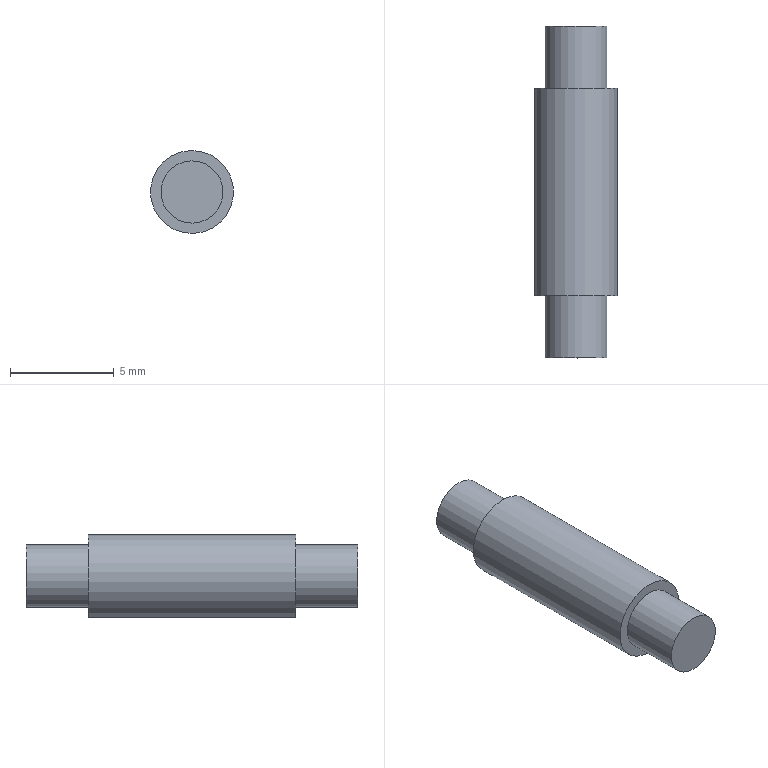Component | NX | CONNECTING_PIN_2_2 | 1 solid | 7 faces | box 4 x 16 x 4 mm | volume 168 mm3 | plane 4 | cylinder 3 | commonest cylinder face diameters 3 x2 4 x1
STEP:
#1=CARTESIAN_POINT('',(0.,0.,0.));
#2=DIRECTION('',(0.,0.,1.));
#3=DIRECTION('',(1.,0.,0.));
#4=AXIS2_PLACEMENT_3D('',#1,#2,#3);
#5=CARTESIAN_POINT('',(-75.879,-51.,18.369));
#6=VERTEX_POINT('',#5);
#7=CARTESIAN_POINT('',(-77.374,-51.,18.5));
#8=DIRECTION('',(0.,-1.,-0.));
#9=DIRECTION('',(0.9962,0.,-0.08716));
#10=AXIS2_PLACEMENT_3D('',#7,#8,#9);
#11=CIRCLE('',#10,1.5);
#12=CARTESIAN_POINT('',(-77.374,-51.,18.5));
#13=DIRECTION('',(0.,1.,0.));
#14=DIRECTION('',(-0.9962,-0.,0.08716));
#15=AXIS2_PLACEMENT_3D('',#12,#13,#14);
#16=PLANE('',#15);
#17=CARTESIAN_POINT('',(-1.5,-0.));
#18=CARTESIAN_POINT('',(-1.5,2.598));
#19=CARTESIAN_POINT('',(0.75,1.299));
#20=CARTESIAN_POINT('',(3.,0.));
#21=CARTESIAN_POINT('',(0.75,-1.299));
#22=CARTESIAN_POINT('',(-1.5,-2.598));
#23=CARTESIAN_POINT('',(-1.5,-0.));
#24=(BOUNDED_CURVE()B_SPLINE_CURVE(2,(#17,#18,#19,#20,#21,#22,#23),.UNSPECIFIED.,.T.,.F.)B_SPLINE_CURVE_WITH_KNOTS((1,2,2,2,2,1),(-2.094,0.,2.094,4.189,6.283,8.378),.UNSPECIFIED.)CURVE()GEOMETRIC_REPRESENTATION_ITEM()RATIONAL_B_SPLINE_CURVE((1.,0.5,1.,0.5,1.,0.5,1.))REPRESENTATION_ITEM(''));
#25=(GEOMETRIC_REPRESENTATION_CONTEXT(2)PARAMETRIC_REPRESENTATION_CONTEXT()REPRESENTATION_CONTEXT('',''));
#26=DEFINITIONAL_REPRESENTATION('',(#24),#25);
#27=PCURVE('',#16,#26);
#28=CARTESIAN_POINT('',(-77.374,-51.,18.5));
#29=DIRECTION('',(0.,-1.,-0.));
#30=DIRECTION('',(0.9962,0.,-0.08716));
#31=AXIS2_PLACEMENT_3D('',#28,#29,#30);
#32=CYLINDRICAL_SURFACE('',#31,1.5);
#33=CARTESIAN_POINT('',(0.,0.));
#34=DIRECTION('',(1.,0.));
#35=VECTOR('',#34,1.);
#36=LINE('',#33,#35);
#37=(GEOMETRIC_REPRESENTATION_CONTEXT(2)PARAMETRIC_REPRESENTATION_CONTEXT()REPRESENTATION_CONTEXT('',''));
#38=DEFINITIONAL_REPRESENTATION('',(#36),#37);
#39=PCURVE('',#32,#38);
#40=SURFACE_CURVE('',#11,(#27,#39),.PCURVE_S1.);
#41=EDGE_CURVE('',#6,#6,#40,.T.);
#42=ORIENTED_EDGE('',*,*,#41,.F.);
#43=EDGE_LOOP('',(#42));
#44=FACE_BOUND('',#43,.T.);
#45=ADVANCED_FACE('',(#44),#16,.T.);
#46=CARTESIAN_POINT('',(-75.879,-54.,18.369));
#47=VERTEX_POINT('',#46);
#48=CARTESIAN_POINT('',(-77.374,-54.,18.5));
#49=DIRECTION('',(-0.,1.,0.));
#50=DIRECTION('',(0.9962,0.,-0.08716));
#51=AXIS2_PLACEMENT_3D('',#48,#49,#50);
#52=CIRCLE('',#51,1.5);
#53=CARTESIAN_POINT('',(6.283,3.));
#54=DIRECTION('',(-1.,0.));
#55=VECTOR('',#54,1.);
#56=LINE('',#53,#55);
#57=(GEOMETRIC_REPRESENTATION_CONTEXT(2)PARAMETRIC_REPRESENTATION_CONTEXT()REPRESENTATION_CONTEXT('',''));
#58=DEFINITIONAL_REPRESENTATION('',(#56),#57);
#59=PCURVE('',#32,#58);
#60=CARTESIAN_POINT('',(-77.374,-54.,18.5));
#61=DIRECTION('',(0.,1.,0.));
#62=DIRECTION('',(-0.9962,-0.,0.08716));
#63=AXIS2_PLACEMENT_3D('',#60,#61,#62);
#64=PLANE('',#63);
#65=CARTESIAN_POINT('',(0.,0.));
#66=DIRECTION('',(-1.,-0.));
#67=AXIS2_PLACEMENT_2D('',#65,#66);
#68=CIRCLE('',#67,1.5);
#69=(GEOMETRIC_REPRESENTATION_CONTEXT(2)PARAMETRIC_REPRESENTATION_CONTEXT()REPRESENTATION_CONTEXT('',''));
#70=DEFINITIONAL_REPRESENTATION('',(#68),#69);
#71=PCURVE('',#64,#70);
#72=SURFACE_CURVE('',#52,(#59,#71),.PCURVE_S1.);
#73=EDGE_CURVE('',#47,#47,#72,.T.);
#74=ORIENTED_EDGE('',*,*,#73,.T.);
#75=CARTESIAN_POINT('',(-75.879,-51.,18.369));
#76=CARTESIAN_POINT('',(-75.879,-54.,18.369));
#77=B_SPLINE_CURVE_WITH_KNOTS('',1,(#75,#76),.UNSPECIFIED.,.F.,.F.,(2,2),(0.,3.),.PIECEWISE_BEZIER_KNOTS.);
#78=CARTESIAN_POINT('',(0.,0.));
#79=DIRECTION('',(0.,1.));
#80=VECTOR('',#79,1.);
#81=LINE('',#78,#80);
#82=(GEOMETRIC_REPRESENTATION_CONTEXT(2)PARAMETRIC_REPRESENTATION_CONTEXT()REPRESENTATION_CONTEXT('',''));
#83=DEFINITIONAL_REPRESENTATION('',(#81),#82);
#84=PCURVE('',#32,#83);
#85=CARTESIAN_POINT('',(6.283,0.));
#86=DIRECTION('',(0.,1.));
#87=VECTOR('',#86,1.);
#88=LINE('',#85,#87);
#89=(GEOMETRIC_REPRESENTATION_CONTEXT(2)PARAMETRIC_REPRESENTATION_CONTEXT()REPRESENTATION_CONTEXT('',''));
#90=DEFINITIONAL_REPRESENTATION('',(#88),#89);
#91=PCURVE('',#32,#90);
#92=SEAM_CURVE('',#77,(#84,#91),.PCURVE_S1.);
#93=EDGE_CURVE('',#6,#47,#92,.T.);
#94=ORIENTED_EDGE('',*,*,#93,.F.);
#95=ORIENTED_EDGE('',*,*,#41,.T.);
#96=ORIENTED_EDGE('',*,*,#93,.T.);
#97=EDGE_LOOP('',(#74,#94,#95,#96));
#98=FACE_BOUND('',#97,.T.);
#99=ADVANCED_FACE('',(#98),#32,.T.);
#100=CARTESIAN_POINT('',(-75.879,-64.,18.369));
#101=VERTEX_POINT('',#100);
#102=CARTESIAN_POINT('',(-77.374,-64.,18.5));
#103=DIRECTION('',(0.,-1.,-0.));
#104=DIRECTION('',(0.9962,0.,-0.08716));
#105=AXIS2_PLACEMENT_3D('',#102,#103,#104);
#106=CIRCLE('',#105,1.5);
#107=CARTESIAN_POINT('',(-77.374,-64.,18.5));
#108=DIRECTION('',(0.,-1.,-0.));
#109=DIRECTION('',(0.9962,0.,-0.08716));
#110=AXIS2_PLACEMENT_3D('',#107,#108,#109);
#111=PLANE('',#110);
#112=CARTESIAN_POINT('',(0.,0.));
#113=DIRECTION('',(1.,-0.));
#114=AXIS2_PLACEMENT_2D('',#112,#113);
#115=CIRCLE('',#114,1.5);
#116=(GEOMETRIC_REPRESENTATION_CONTEXT(2)PARAMETRIC_REPRESENTATION_CONTEXT()REPRESENTATION_CONTEXT('',''));
#117=DEFINITIONAL_REPRESENTATION('',(#115),#116);
#118=PCURVE('',#111,#117);
#119=CARTESIAN_POINT('',(-77.374,-64.,18.5));
#120=DIRECTION('',(0.,-1.,-0.));
#121=DIRECTION('',(0.9962,0.,-0.08716));
#122=AXIS2_PLACEMENT_3D('',#119,#120,#121);
#123=CYLINDRICAL_SURFACE('',#122,1.5);
#124=CARTESIAN_POINT('',(0.,0.));
#125=DIRECTION('',(1.,0.));
#126=VECTOR('',#125,1.);
#127=LINE('',#124,#126);
#128=(GEOMETRIC_REPRESENTATION_CONTEXT(2)PARAMETRIC_REPRESENTATION_CONTEXT()REPRESENTATION_CONTEXT('',''));
#129=DEFINITIONAL_REPRESENTATION('',(#127),#128);
#130=PCURVE('',#123,#129);
#131=SURFACE_CURVE('',#106,(#118,#130),.PCURVE_S1.);
#132=EDGE_CURVE('',#101,#101,#131,.T.);
#133=ORIENTED_EDGE('',*,*,#132,.F.);
#134=EDGE_LOOP('',(#133));
#135=FACE_BOUND('',#134,.T.);
#136=CARTESIAN_POINT('',(-75.381,-64.,18.326));
#137=VERTEX_POINT('',#136);
#138=CARTESIAN_POINT('',(-77.374,-64.,18.5));
#139=DIRECTION('',(0.,-1.,-0.));
#140=DIRECTION('',(0.9962,0.,-0.08716));
#141=AXIS2_PLACEMENT_3D('',#138,#139,#140);
#142=CIRCLE('',#141,2.);
#143=CARTESIAN_POINT('',(0.,0.));
#144=DIRECTION('',(1.,-0.));
#145=AXIS2_PLACEMENT_2D('',#143,#144);
#146=CIRCLE('',#145,2.);
#147=(GEOMETRIC_REPRESENTATION_CONTEXT(2)PARAMETRIC_REPRESENTATION_CONTEXT()REPRESENTATION_CONTEXT('',''));
#148=DEFINITIONAL_REPRESENTATION('',(#146),#147);
#149=PCURVE('',#111,#148);
#150=CARTESIAN_POINT('',(-77.374,-54.,18.5));
#151=DIRECTION('',(0.,-1.,-0.));
#152=DIRECTION('',(0.9962,0.,-0.08716));
#153=AXIS2_PLACEMENT_3D('',#150,#151,#152);
#154=CYLINDRICAL_SURFACE('',#153,2.);
#155=CARTESIAN_POINT('',(0.,10.));
#156=DIRECTION('',(1.,0.));
#157=VECTOR('',#156,1.);
#158=LINE('',#155,#157);
#159=(GEOMETRIC_REPRESENTATION_CONTEXT(2)PARAMETRIC_REPRESENTATION_CONTEXT()REPRESENTATION_CONTEXT('',''));
#160=DEFINITIONAL_REPRESENTATION('',(#158),#159);
#161=PCURVE('',#154,#160);
#162=SURFACE_CURVE('',#142,(#149,#161),.PCURVE_S1.);
#163=EDGE_CURVE('',#137,#137,#162,.T.);
#164=ORIENTED_EDGE('',*,*,#163,.T.);
#165=EDGE_LOOP('',(#164));
#166=FACE_BOUND('',#165,.T.);
#167=ADVANCED_FACE('',(#135,#166),#111,.T.);
#168=ORIENTED_EDGE('',*,*,#73,.F.);
#169=EDGE_LOOP('',(#168));
#170=FACE_BOUND('',#169,.T.);
#171=CARTESIAN_POINT('',(-75.381,-54.,18.326));
#172=VERTEX_POINT('',#171);
#173=CARTESIAN_POINT('',(-77.374,-54.,18.5));
#174=DIRECTION('',(0.,-1.,-0.));
#175=DIRECTION('',(0.9962,0.,-0.08716));
#176=AXIS2_PLACEMENT_3D('',#173,#174,#175);
#177=CIRCLE('',#176,2.);
#178=CARTESIAN_POINT('',(-2.,-0.));
#179=CARTESIAN_POINT('',(-2.,3.464));
#180=CARTESIAN_POINT('',(1.,1.732));
#181=CARTESIAN_POINT('',(4.,0.));
#182=CARTESIAN_POINT('',(1.,-1.732));
#183=CARTESIAN_POINT('',(-2.,-3.464));
#184=CARTESIAN_POINT('',(-2.,-0.));
#185=(BOUNDED_CURVE()B_SPLINE_CURVE(2,(#178,#179,#180,#181,#182,#183,#184),.UNSPECIFIED.,.T.,.F.)B_SPLINE_CURVE_WITH_KNOTS((1,2,2,2,2,1),(-2.094,0.,2.094,4.189,6.283,8.378),.UNSPECIFIED.)CURVE()GEOMETRIC_REPRESENTATION_ITEM()RATIONAL_B_SPLINE_CURVE((1.,0.5,1.,0.5,1.,0.5,1.))REPRESENTATION_ITEM(''));
#186=(GEOMETRIC_REPRESENTATION_CONTEXT(2)PARAMETRIC_REPRESENTATION_CONTEXT()REPRESENTATION_CONTEXT('',''));
#187=DEFINITIONAL_REPRESENTATION('',(#185),#186);
#188=PCURVE('',#64,#187);
#189=CARTESIAN_POINT('',(0.,0.));
#190=DIRECTION('',(1.,0.));
#191=VECTOR('',#190,1.);
#192=LINE('',#189,#191);
#193=(GEOMETRIC_REPRESENTATION_CONTEXT(2)PARAMETRIC_REPRESENTATION_CONTEXT()REPRESENTATION_CONTEXT('',''));
#194=DEFINITIONAL_REPRESENTATION('',(#192),#193);
#195=PCURVE('',#154,#194);
#196=SURFACE_CURVE('',#177,(#188,#195),.PCURVE_S1.);
#197=EDGE_CURVE('',#172,#172,#196,.T.);
#198=ORIENTED_EDGE('',*,*,#197,.F.);
#199=EDGE_LOOP('',(#198));
#200=FACE_BOUND('',#199,.T.);
#201=ADVANCED_FACE('',(#170,#200),#64,.T.);
#202=ORIENTED_EDGE('',*,*,#163,.F.);
#203=CARTESIAN_POINT('',(-75.381,-54.,18.326));
#204=CARTESIAN_POINT('',(-75.381,-64.,18.326));
#205=B_SPLINE_CURVE_WITH_KNOTS('',1,(#203,#204),.UNSPECIFIED.,.F.,.F.,(2,2),(0.,10.),.PIECEWISE_BEZIER_KNOTS.);
#206=CARTESIAN_POINT('',(0.,0.));
#207=DIRECTION('',(0.,1.));
#208=VECTOR('',#207,1.);
#209=LINE('',#206,#208);
#210=(GEOMETRIC_REPRESENTATION_CONTEXT(2)PARAMETRIC_REPRESENTATION_CONTEXT()REPRESENTATION_CONTEXT('',''));
#211=DEFINITIONAL_REPRESENTATION('',(#209),#210);
#212=PCURVE('',#154,#211);
#213=CARTESIAN_POINT('',(6.283,0.));
#214=DIRECTION('',(0.,1.));
#215=VECTOR('',#214,1.);
#216=LINE('',#213,#215);
#217=(GEOMETRIC_REPRESENTATION_CONTEXT(2)PARAMETRIC_REPRESENTATION_CONTEXT()REPRESENTATION_CONTEXT('',''));
#218=DEFINITIONAL_REPRESENTATION('',(#216),#217);
#219=PCURVE('',#154,#218);
#220=SEAM_CURVE('',#205,(#212,#219),.PCURVE_S1.);
#221=EDGE_CURVE('',#172,#137,#220,.T.);
#222=ORIENTED_EDGE('',*,*,#221,.F.);
#223=ORIENTED_EDGE('',*,*,#197,.T.);
#224=ORIENTED_EDGE('',*,*,#221,.T.);
#225=EDGE_LOOP('',(#202,#222,#223,#224));
#226=FACE_BOUND('',#225,.T.);
#227=ADVANCED_FACE('',(#226),#154,.T.);
#228=CARTESIAN_POINT('',(-75.879,-67.,18.369));
#229=VERTEX_POINT('',#228);
#230=CARTESIAN_POINT('',(-77.374,-67.,18.5));
#231=DIRECTION('',(0.,-1.,-0.));
#232=DIRECTION('',(0.9962,0.,-0.08716));
#233=AXIS2_PLACEMENT_3D('',#230,#231,#232);
#234=CIRCLE('',#233,1.5);
#235=CARTESIAN_POINT('',(-77.374,-67.,18.5));
#236=DIRECTION('',(0.,-1.,-0.));
#237=DIRECTION('',(0.9962,0.,-0.08716));
#238=AXIS2_PLACEMENT_3D('',#235,#236,#237);
#239=PLANE('',#238);
#240=CARTESIAN_POINT('',(0.,0.));
#241=DIRECTION('',(1.,-0.));
#242=AXIS2_PLACEMENT_2D('',#240,#241);
#243=CIRCLE('',#242,1.5);
#244=(GEOMETRIC_REPRESENTATION_CONTEXT(2)PARAMETRIC_REPRESENTATION_CONTEXT()REPRESENTATION_CONTEXT('',''));
#245=DEFINITIONAL_REPRESENTATION('',(#243),#244);
#246=PCURVE('',#239,#245);
#247=CARTESIAN_POINT('',(0.,3.));
#248=DIRECTION('',(1.,0.));
#249=VECTOR('',#248,1.);
#250=LINE('',#247,#249);
#251=(GEOMETRIC_REPRESENTATION_CONTEXT(2)PARAMETRIC_REPRESENTATION_CONTEXT()REPRESENTATION_CONTEXT('',''));
#252=DEFINITIONAL_REPRESENTATION('',(#250),#251);
#253=PCURVE('',#123,#252);
#254=SURFACE_CURVE('',#234,(#246,#253),.PCURVE_S1.);
#255=EDGE_CURVE('',#229,#229,#254,.T.);
#256=ORIENTED_EDGE('',*,*,#255,.T.);
#257=EDGE_LOOP('',(#256));
#258=FACE_BOUND('',#257,.T.);
#259=ADVANCED_FACE('',(#258),#239,.T.);
#260=ORIENTED_EDGE('',*,*,#255,.F.);
#261=CARTESIAN_POINT('',(-75.879,-64.,18.369));
#262=CARTESIAN_POINT('',(-75.879,-67.,18.369));
#263=B_SPLINE_CURVE_WITH_KNOTS('',1,(#261,#262),.UNSPECIFIED.,.F.,.F.,(2,2),(0.,3.),.PIECEWISE_BEZIER_KNOTS.);
#264=CARTESIAN_POINT('',(0.,0.));
#265=DIRECTION('',(0.,1.));
#266=VECTOR('',#265,1.);
#267=LINE('',#264,#266);
#268=(GEOMETRIC_REPRESENTATION_CONTEXT(2)PARAMETRIC_REPRESENTATION_CONTEXT()REPRESENTATION_CONTEXT('',''));
#269=DEFINITIONAL_REPRESENTATION('',(#267),#268);
#270=PCURVE('',#123,#269);
#271=CARTESIAN_POINT('',(6.283,0.));
#272=DIRECTION('',(0.,1.));
#273=VECTOR('',#272,1.);
#274=LINE('',#271,#273);
#275=(GEOMETRIC_REPRESENTATION_CONTEXT(2)PARAMETRIC_REPRESENTATION_CONTEXT()REPRESENTATION_CONTEXT('',''));
#276=DEFINITIONAL_REPRESENTATION('',(#274),#275);
#277=PCURVE('',#123,#276);
#278=SEAM_CURVE('',#263,(#270,#277),.PCURVE_S1.);
#279=EDGE_CURVE('',#101,#229,#278,.T.);
#280=ORIENTED_EDGE('',*,*,#279,.F.);
#281=ORIENTED_EDGE('',*,*,#132,.T.);
#282=ORIENTED_EDGE('',*,*,#279,.T.);
#283=EDGE_LOOP('',(#260,#280,#281,#282));
#284=FACE_BOUND('',#283,.T.);
#285=ADVANCED_FACE('',(#284),#123,.T.);
#286=CLOSED_SHELL('',(#45,#99,#167,#201,#227,#259,#285));
#287=MANIFOLD_SOLID_BREP('',#286);
#288=(LENGTH_UNIT()NAMED_UNIT(*)SI_UNIT(.MILLI.,.METRE.));
#289=UNCERTAINTY_MEASURE_WITH_UNIT(LENGTH_MEASURE(0.00001),#288,'','');
#290=(NAMED_UNIT(*)PLANE_ANGLE_UNIT()SI_UNIT($,.RADIAN.));
#291=(NAMED_UNIT(*)SI_UNIT($,.STERADIAN.)SOLID_ANGLE_UNIT());
#292=(GEOMETRIC_REPRESENTATION_CONTEXT(3)GLOBAL_UNCERTAINTY_ASSIGNED_CONTEXT((#289))GLOBAL_UNIT_ASSIGNED_CONTEXT((#288,#290,#291))REPRESENTATION_CONTEXT('',''));
#293=ADVANCED_BREP_SHAPE_REPRESENTATION('',(#4,#287),#292);